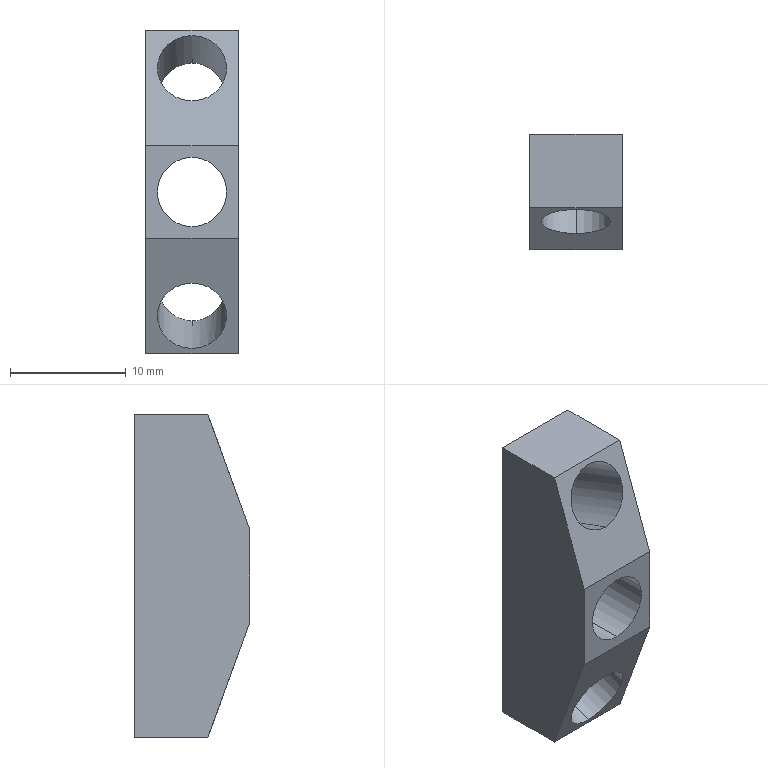Component | SolidWorks | ConnectingBlock-1 | 1 solid | 14 faces | box 8 x 10 x 28 mm | volume 1211 mm3 | plane 8 | cylinder 6 | commonest cylinder face diameters 6 x6
STEP:
#1=CARTESIAN_POINT('',(-5.544,0.8852,39.537));
#2=VERTEX_POINT('',#1);
#3=CARTESIAN_POINT('',(-5.544,0.8852,39.285));
#4=VERTEX_POINT('',#3);
#5=CARTESIAN_POINT('',(-5.544,0.8852,39.537));
#6=CARTESIAN_POINT('',(-5.308,0.8852,39.537));
#7=CARTESIAN_POINT('',(-5.308,0.8852,39.285));
#8=CARTESIAN_POINT('',(-5.544,0.8852,39.285));
#9=(BOUNDED_CURVE()B_SPLINE_CURVE(3,(#5,#6,#7,#8),.UNSPECIFIED.,.F.,.F.)B_SPLINE_CURVE_WITH_KNOTS((4,4),(3.142,6.283),.UNSPECIFIED.)CURVE()GEOMETRIC_REPRESENTATION_ITEM()RATIONAL_B_SPLINE_CURVE((1.,0.3333,0.3333,1.))REPRESENTATION_ITEM(''));
#10=EDGE_CURVE('',#2,#4,#9,.T.);
#11=ORIENTED_EDGE('',*,*,#10,.T.);
#12=CARTESIAN_POINT('',(-5.544,0.628,39.192));
#13=VERTEX_POINT('',#12);
#14=CARTESIAN_POINT('',(-5.544,1.109,39.367));
#15=DIRECTION('',(-0.,-0.9397,-0.342));
#16=VECTOR('',#15,39.37);
#17=LINE('',#14,#16);
#18=EDGE_CURVE('',#4,#13,#17,.T.);
#19=ORIENTED_EDGE('',*,*,#18,.T.);
#20=CARTESIAN_POINT('',(-5.544,0.5472,39.414));
#21=VERTEX_POINT('',#20);
#22=CARTESIAN_POINT('',(-5.544,0.5876,39.303));
#23=DIRECTION('',(0.,0.9397,0.342));
#24=DIRECTION('',(0.,0.342,-0.9397));
#25=AXIS2_PLACEMENT_3D('',#22,#23,#24);
#26=CIRCLE('',#25,0.1181);
#27=EDGE_CURVE('',#21,#13,#26,.T.);
#28=ORIENTED_EDGE('',*,*,#27,.F.);
#29=CARTESIAN_POINT('',(-5.544,1.028,39.589));
#30=DIRECTION('',(-0.,-0.9397,-0.342));
#31=VECTOR('',#30,39.37);
#32=LINE('',#29,#31);
#33=EDGE_CURVE('',#2,#21,#32,.T.);
#34=ORIENTED_EDGE('',*,*,#33,.F.);
#35=EDGE_LOOP('',(#11,#19,#28,#34));
#36=FACE_OUTER_BOUND('',#35,.T.);
#37=CARTESIAN_POINT('',(-5.544,1.069,39.478));
#38=DIRECTION('',(-0.,-0.9397,-0.342));
#39=DIRECTION('',(0.,-0.342,0.9397));
#40=AXIS2_PLACEMENT_3D('',#37,#38,#39);
#41=CYLINDRICAL_SURFACE('',#40,0.1181);
#42=ADVANCED_FACE('',(#36),#41,.F.);
#43=CARTESIAN_POINT('',(-5.544,0.8852,39.912));
#44=VERTEX_POINT('',#43);
#45=CARTESIAN_POINT('',(-5.544,0.8852,40.164));
#46=VERTEX_POINT('',#45);
#47=CARTESIAN_POINT('',(-5.544,0.8852,39.912));
#48=CARTESIAN_POINT('',(-5.308,0.8852,39.912));
#49=CARTESIAN_POINT('',(-5.308,0.8852,40.164));
#50=CARTESIAN_POINT('',(-5.544,0.8852,40.164));
#51=(BOUNDED_CURVE()B_SPLINE_CURVE(3,(#47,#48,#49,#50),.UNSPECIFIED.,.F.,.F.)B_SPLINE_CURVE_WITH_KNOTS((4,4),(3.142,6.283),.UNSPECIFIED.)CURVE()GEOMETRIC_REPRESENTATION_ITEM()RATIONAL_B_SPLINE_CURVE((1.,0.3333,0.3333,1.))REPRESENTATION_ITEM(''));
#52=EDGE_CURVE('',#44,#46,#51,.T.);
#53=ORIENTED_EDGE('',*,*,#52,.F.);
#54=CARTESIAN_POINT('',(-5.544,0.5472,40.035));
#55=VERTEX_POINT('',#54);
#56=CARTESIAN_POINT('',(-5.544,1.028,39.86));
#57=DIRECTION('',(-0.,-0.9397,0.342));
#58=VECTOR('',#57,39.37);
#59=LINE('',#56,#58);
#60=EDGE_CURVE('',#44,#55,#59,.T.);
#61=ORIENTED_EDGE('',*,*,#60,.T.);
#62=CARTESIAN_POINT('',(-5.544,0.628,40.257));
#63=VERTEX_POINT('',#62);
#64=CARTESIAN_POINT('',(-5.544,0.5876,40.146));
#65=DIRECTION('',(-0.,-0.9397,0.342));
#66=DIRECTION('',(0.,0.342,0.9397));
#67=AXIS2_PLACEMENT_3D('',#64,#65,#66);
#68=CIRCLE('',#67,0.1181);
#69=EDGE_CURVE('',#55,#63,#68,.T.);
#70=ORIENTED_EDGE('',*,*,#69,.T.);
#71=CARTESIAN_POINT('',(-5.544,1.109,40.082));
#72=DIRECTION('',(-0.,-0.9397,0.342));
#73=VECTOR('',#72,39.37);
#74=LINE('',#71,#73);
#75=EDGE_CURVE('',#46,#63,#74,.T.);
#76=ORIENTED_EDGE('',*,*,#75,.F.);
#77=EDGE_LOOP('',(#53,#61,#70,#76));
#78=FACE_OUTER_BOUND('',#77,.T.);
#79=CARTESIAN_POINT('',(-5.544,1.069,39.971));
#80=DIRECTION('',(-0.,-0.9397,0.342));
#81=DIRECTION('',(0.,0.342,0.9397));
#82=AXIS2_PLACEMENT_3D('',#79,#80,#81);
#83=CYLINDRICAL_SURFACE('',#82,0.1181);
#84=ADVANCED_FACE('',(#78),#83,.F.);
#85=CARTESIAN_POINT('',(-5.544,0.8852,39.606));
#86=VERTEX_POINT('',#85);
#87=CARTESIAN_POINT('',(-5.544,0.8852,39.843));
#88=VERTEX_POINT('',#87);
#89=CARTESIAN_POINT('',(-5.544,0.8852,39.724));
#90=DIRECTION('',(-0.,-1.,0.));
#91=DIRECTION('',(0.,0.,1.));
#92=AXIS2_PLACEMENT_3D('',#89,#90,#91);
#93=CIRCLE('',#92,0.1181);
#94=EDGE_CURVE('',#86,#88,#93,.T.);
#95=ORIENTED_EDGE('',*,*,#94,.F.);
#96=CARTESIAN_POINT('',(-5.544,0.4915,39.606));
#97=VERTEX_POINT('',#96);
#98=CARTESIAN_POINT('',(-5.544,1.003,39.606));
#99=DIRECTION('',(-0.,-1.,0.));
#100=VECTOR('',#99,39.37);
#101=LINE('',#98,#100);
#102=EDGE_CURVE('',#86,#97,#101,.T.);
#103=ORIENTED_EDGE('',*,*,#102,.T.);
#104=CARTESIAN_POINT('',(-5.544,0.4915,39.843));
#105=VERTEX_POINT('',#104);
#106=CARTESIAN_POINT('',(-5.544,0.4915,39.724));
#107=DIRECTION('',(-0.,-1.,0.));
#108=DIRECTION('',(0.,0.,1.));
#109=AXIS2_PLACEMENT_3D('',#106,#107,#108);
#110=CIRCLE('',#109,0.1181);
#111=EDGE_CURVE('',#97,#105,#110,.T.);
#112=ORIENTED_EDGE('',*,*,#111,.T.);
#113=CARTESIAN_POINT('',(-5.544,1.003,39.843));
#114=DIRECTION('',(-0.,-1.,0.));
#115=VECTOR('',#114,39.37);
#116=LINE('',#113,#115);
#117=EDGE_CURVE('',#88,#105,#116,.T.);
#118=ORIENTED_EDGE('',*,*,#117,.F.);
#119=EDGE_LOOP('',(#95,#103,#112,#118));
#120=FACE_OUTER_BOUND('',#119,.T.);
#121=CARTESIAN_POINT('',(-5.544,1.003,39.724));
#122=DIRECTION('',(-0.,-1.,0.));
#123=DIRECTION('',(0.,0.,1.));
#124=AXIS2_PLACEMENT_3D('',#121,#122,#123);
#125=CYLINDRICAL_SURFACE('',#124,0.1181);
#126=ADVANCED_FACE('',(#120),#125,.F.);
#127=CARTESIAN_POINT('',(-5.387,0.8852,39.173));
#128=VERTEX_POINT('',#127);
#129=CARTESIAN_POINT('',(-5.387,0.6348,39.173));
#130=VERTEX_POINT('',#129);
#131=CARTESIAN_POINT('',(-5.387,0.6348,39.173));
#132=DIRECTION('',(-0.,-1.,0.));
#133=VECTOR('',#132,39.37);
#134=LINE('',#131,#133);
#135=EDGE_CURVE('',#128,#130,#134,.T.);
#136=ORIENTED_EDGE('',*,*,#135,.T.);
#137=CARTESIAN_POINT('',(-5.701,0.6348,39.173));
#138=VERTEX_POINT('',#137);
#139=CARTESIAN_POINT('',(-5.701,0.6348,39.173));
#140=DIRECTION('',(1.,-0.,-0.));
#141=VECTOR('',#140,39.37);
#142=LINE('',#139,#141);
#143=EDGE_CURVE('',#138,#130,#142,.T.);
#144=ORIENTED_EDGE('',*,*,#143,.F.);
#145=CARTESIAN_POINT('',(-5.701,0.8852,39.173));
#146=VERTEX_POINT('',#145);
#147=CARTESIAN_POINT('',(-5.701,0.6348,39.173));
#148=DIRECTION('',(-0.,-1.,0.));
#149=VECTOR('',#148,39.37);
#150=LINE('',#147,#149);
#151=EDGE_CURVE('',#146,#138,#150,.T.);
#152=ORIENTED_EDGE('',*,*,#151,.F.);
#153=CARTESIAN_POINT('',(-5.701,0.8852,39.173));
#154=DIRECTION('',(1.,-0.,-0.));
#155=VECTOR('',#154,39.37);
#156=LINE('',#153,#155);
#157=EDGE_CURVE('',#146,#128,#156,.T.);
#158=ORIENTED_EDGE('',*,*,#157,.T.);
#159=EDGE_LOOP('',(#136,#144,#152,#158));
#160=FACE_OUTER_BOUND('',#159,.T.);
#161=CARTESIAN_POINT('',(-5.701,0.6348,39.173));
#162=DIRECTION('',(0.,0.,1.));
#163=DIRECTION('',(0.,1.,-0.));
#164=AXIS2_PLACEMENT_3D('',#161,#162,#163);
#165=PLANE('',#164);
#166=ADVANCED_FACE('',(#160),#165,.F.);
#167=ORIENTED_EDGE('',*,*,#27,.T.);
#168=CARTESIAN_POINT('',(-5.544,0.5876,39.303));
#169=DIRECTION('',(0.,0.9397,0.342));
#170=DIRECTION('',(0.,0.342,-0.9397));
#171=AXIS2_PLACEMENT_3D('',#168,#169,#170);
#172=CIRCLE('',#171,0.1181);
#173=EDGE_CURVE('',#13,#21,#172,.T.);
#174=ORIENTED_EDGE('',*,*,#173,.T.);
#175=EDGE_LOOP('',(#167,#174));
#176=FACE_BOUND('',#175,.T.);
#177=CARTESIAN_POINT('',(-5.387,0.4915,39.567));
#178=VERTEX_POINT('',#177);
#179=CARTESIAN_POINT('',(-5.387,0.4915,39.567));
#180=DIRECTION('',(0.,-0.342,0.9397));
#181=VECTOR('',#180,39.37);
#182=LINE('',#179,#181);
#183=EDGE_CURVE('',#130,#178,#182,.T.);
#184=ORIENTED_EDGE('',*,*,#183,.T.);
#185=CARTESIAN_POINT('',(-5.701,0.4915,39.567));
#186=VERTEX_POINT('',#185);
#187=CARTESIAN_POINT('',(-5.701,0.4915,39.567));
#188=DIRECTION('',(1.,-0.,-0.));
#189=VECTOR('',#188,39.37);
#190=LINE('',#187,#189);
#191=EDGE_CURVE('',#186,#178,#190,.T.);
#192=ORIENTED_EDGE('',*,*,#191,.F.);
#193=CARTESIAN_POINT('',(-5.701,0.4915,39.567));
#194=DIRECTION('',(0.,-0.342,0.9397));
#195=VECTOR('',#194,39.37);
#196=LINE('',#193,#195);
#197=EDGE_CURVE('',#138,#186,#196,.T.);
#198=ORIENTED_EDGE('',*,*,#197,.F.);
#199=ORIENTED_EDGE('',*,*,#143,.T.);
#200=EDGE_LOOP('',(#184,#192,#198,#199));
#201=FACE_OUTER_BOUND('',#200,.T.);
#202=CARTESIAN_POINT('',(-5.701,0.4915,39.567));
#203=DIRECTION('',(0.,0.9397,0.342));
#204=DIRECTION('',(-0.,0.342,-0.9397));
#205=AXIS2_PLACEMENT_3D('',#202,#203,#204);
#206=PLANE('',#205);
#207=ADVANCED_FACE('',(#176,#201),#206,.F.);
#208=CARTESIAN_POINT('',(-5.544,0.4915,39.724));
#209=DIRECTION('',(-0.,-1.,0.));
#210=DIRECTION('',(0.,0.,1.));
#211=AXIS2_PLACEMENT_3D('',#208,#209,#210);
#212=CIRCLE('',#211,0.1181);
#213=EDGE_CURVE('',#105,#97,#212,.T.);
#214=ORIENTED_EDGE('',*,*,#213,.F.);
#215=ORIENTED_EDGE('',*,*,#111,.F.);
#216=EDGE_LOOP('',(#214,#215));
#217=FACE_BOUND('',#216,.T.);
#218=CARTESIAN_POINT('',(-5.387,0.4915,39.882));
#219=VERTEX_POINT('',#218);
#220=CARTESIAN_POINT('',(-5.387,0.4915,39.882));
#221=DIRECTION('',(0.,0.,1.));
#222=VECTOR('',#221,39.37);
#223=LINE('',#220,#222);
#224=EDGE_CURVE('',#178,#219,#223,.T.);
#225=ORIENTED_EDGE('',*,*,#224,.T.);
#226=CARTESIAN_POINT('',(-5.701,0.4915,39.882));
#227=VERTEX_POINT('',#226);
#228=CARTESIAN_POINT('',(-5.701,0.4915,39.882));
#229=DIRECTION('',(1.,-0.,-0.));
#230=VECTOR('',#229,39.37);
#231=LINE('',#228,#230);
#232=EDGE_CURVE('',#227,#219,#231,.T.);
#233=ORIENTED_EDGE('',*,*,#232,.F.);
#234=CARTESIAN_POINT('',(-5.701,0.4915,39.882));
#235=DIRECTION('',(0.,0.,1.));
#236=VECTOR('',#235,39.37);
#237=LINE('',#234,#236);
#238=EDGE_CURVE('',#186,#227,#237,.T.);
#239=ORIENTED_EDGE('',*,*,#238,.F.);
#240=ORIENTED_EDGE('',*,*,#191,.T.);
#241=EDGE_LOOP('',(#225,#233,#239,#240));
#242=FACE_OUTER_BOUND('',#241,.T.);
#243=CARTESIAN_POINT('',(-5.701,0.4915,39.882));
#244=DIRECTION('',(0.,1.,-0.));
#245=DIRECTION('',(-0.,-0.,-1.));
#246=AXIS2_PLACEMENT_3D('',#243,#244,#245);
#247=PLANE('',#246);
#248=ADVANCED_FACE('',(#217,#242),#247,.F.);
#249=CARTESIAN_POINT('',(-5.544,0.5876,40.146));
#250=DIRECTION('',(-0.,-0.9397,0.342));
#251=DIRECTION('',(0.,0.342,0.9397));
#252=AXIS2_PLACEMENT_3D('',#249,#250,#251);
#253=CIRCLE('',#252,0.1181);
#254=EDGE_CURVE('',#63,#55,#253,.T.);
#255=ORIENTED_EDGE('',*,*,#254,.F.);
#256=ORIENTED_EDGE('',*,*,#69,.F.);
#257=EDGE_LOOP('',(#255,#256));
#258=FACE_BOUND('',#257,.T.);
#259=CARTESIAN_POINT('',(-5.387,0.6348,40.276));
#260=VERTEX_POINT('',#259);
#261=CARTESIAN_POINT('',(-5.387,0.6348,40.276));
#262=DIRECTION('',(0.,0.342,0.9397));
#263=VECTOR('',#262,39.37);
#264=LINE('',#261,#263);
#265=EDGE_CURVE('',#219,#260,#264,.T.);
#266=ORIENTED_EDGE('',*,*,#265,.T.);
#267=CARTESIAN_POINT('',(-5.701,0.6348,40.276));
#268=VERTEX_POINT('',#267);
#269=CARTESIAN_POINT('',(-5.701,0.6348,40.276));
#270=DIRECTION('',(1.,-0.,-0.));
#271=VECTOR('',#270,39.37);
#272=LINE('',#269,#271);
#273=EDGE_CURVE('',#268,#260,#272,.T.);
#274=ORIENTED_EDGE('',*,*,#273,.F.);
#275=CARTESIAN_POINT('',(-5.701,0.6348,40.276));
#276=DIRECTION('',(0.,0.342,0.9397));
#277=VECTOR('',#276,39.37);
#278=LINE('',#275,#277);
#279=EDGE_CURVE('',#227,#268,#278,.T.);
#280=ORIENTED_EDGE('',*,*,#279,.F.);
#281=ORIENTED_EDGE('',*,*,#232,.T.);
#282=EDGE_LOOP('',(#266,#274,#280,#281));
#283=FACE_OUTER_BOUND('',#282,.T.);
#284=CARTESIAN_POINT('',(-5.701,0.6348,40.276));
#285=DIRECTION('',(0.,0.9397,-0.342));
#286=DIRECTION('',(-0.,-0.342,-0.9397));
#287=AXIS2_PLACEMENT_3D('',#284,#285,#286);
#288=PLANE('',#287);
#289=ADVANCED_FACE('',(#258,#283),#288,.F.);
#290=CARTESIAN_POINT('',(-5.387,0.8852,40.276));
#291=VERTEX_POINT('',#290);
#292=CARTESIAN_POINT('',(-5.387,0.8852,40.276));
#293=DIRECTION('',(0.,1.,-0.));
#294=VECTOR('',#293,39.37);
#295=LINE('',#292,#294);
#296=EDGE_CURVE('',#260,#291,#295,.T.);
#297=ORIENTED_EDGE('',*,*,#296,.T.);
#298=CARTESIAN_POINT('',(-5.701,0.8852,40.276));
#299=VERTEX_POINT('',#298);
#300=CARTESIAN_POINT('',(-5.701,0.8852,40.276));
#301=DIRECTION('',(1.,-0.,-0.));
#302=VECTOR('',#301,39.37);
#303=LINE('',#300,#302);
#304=EDGE_CURVE('',#299,#291,#303,.T.);
#305=ORIENTED_EDGE('',*,*,#304,.F.);
#306=CARTESIAN_POINT('',(-5.701,0.8852,40.276));
#307=DIRECTION('',(0.,1.,-0.));
#308=VECTOR('',#307,39.37);
#309=LINE('',#306,#308);
#310=EDGE_CURVE('',#268,#299,#309,.T.);
#311=ORIENTED_EDGE('',*,*,#310,.F.);
#312=ORIENTED_EDGE('',*,*,#273,.T.);
#313=EDGE_LOOP('',(#297,#305,#311,#312));
#314=FACE_OUTER_BOUND('',#313,.T.);
#315=CARTESIAN_POINT('',(-5.701,0.8852,40.276));
#316=DIRECTION('',(-0.,-0.,-1.));
#317=DIRECTION('',(1.,-0.,-0.));
#318=AXIS2_PLACEMENT_3D('',#315,#316,#317);
#319=PLANE('',#318);
#320=ADVANCED_FACE('',(#314),#319,.F.);
#321=ORIENTED_EDGE('',*,*,#10,.F.);
#322=CARTESIAN_POINT('',(-5.544,0.8852,39.285));
#323=CARTESIAN_POINT('',(-5.78,0.8852,39.285));
#324=CARTESIAN_POINT('',(-5.78,0.8852,39.537));
#325=CARTESIAN_POINT('',(-5.544,0.8852,39.537));
#326=(BOUNDED_CURVE()B_SPLINE_CURVE(3,(#322,#323,#324,#325),.UNSPECIFIED.,.F.,.F.)B_SPLINE_CURVE_WITH_KNOTS((4,4),(0.,3.142),.UNSPECIFIED.)CURVE()GEOMETRIC_REPRESENTATION_ITEM()RATIONAL_B_SPLINE_CURVE((1.,0.3333,0.3333,1.))REPRESENTATION_ITEM(''));
#327=EDGE_CURVE('',#4,#2,#326,.T.);
#328=ORIENTED_EDGE('',*,*,#327,.F.);
#329=EDGE_LOOP('',(#321,#328));
#330=FACE_BOUND('',#329,.T.);
#331=CARTESIAN_POINT('',(-5.544,0.8852,40.164));
#332=CARTESIAN_POINT('',(-5.78,0.8852,40.164));
#333=CARTESIAN_POINT('',(-5.78,0.8852,39.912));
#334=CARTESIAN_POINT('',(-5.544,0.8852,39.912));
#335=(BOUNDED_CURVE()B_SPLINE_CURVE(3,(#331,#332,#333,#334),.UNSPECIFIED.,.F.,.F.)B_SPLINE_CURVE_WITH_KNOTS((4,4),(0.,3.142),.UNSPECIFIED.)CURVE()GEOMETRIC_REPRESENTATION_ITEM()RATIONAL_B_SPLINE_CURVE((1.,0.3333,0.3333,1.))REPRESENTATION_ITEM(''));
#336=EDGE_CURVE('',#46,#44,#335,.T.);
#337=ORIENTED_EDGE('',*,*,#336,.T.);
#338=ORIENTED_EDGE('',*,*,#52,.T.);
#339=EDGE_LOOP('',(#337,#338));
#340=FACE_BOUND('',#339,.T.);
#341=CARTESIAN_POINT('',(-5.544,0.8852,39.724));
#342=DIRECTION('',(-0.,-1.,0.));
#343=DIRECTION('',(0.,0.,1.));
#344=AXIS2_PLACEMENT_3D('',#341,#342,#343);
#345=CIRCLE('',#344,0.1181);
#346=EDGE_CURVE('',#88,#86,#345,.T.);
#347=ORIENTED_EDGE('',*,*,#346,.T.);
#348=ORIENTED_EDGE('',*,*,#94,.T.);
#349=EDGE_LOOP('',(#347,#348));
#350=FACE_BOUND('',#349,.T.);
#351=CARTESIAN_POINT('',(-5.387,0.8852,40.276));
#352=DIRECTION('',(-0.,-0.,-1.));
#353=VECTOR('',#352,39.37);
#354=LINE('',#351,#353);
#355=EDGE_CURVE('',#291,#128,#354,.T.);
#356=ORIENTED_EDGE('',*,*,#355,.T.);
#357=ORIENTED_EDGE('',*,*,#157,.F.);
#358=CARTESIAN_POINT('',(-5.701,0.8852,40.276));
#359=DIRECTION('',(-0.,-0.,-1.));
#360=VECTOR('',#359,39.37);
#361=LINE('',#358,#360);
#362=EDGE_CURVE('',#299,#146,#361,.T.);
#363=ORIENTED_EDGE('',*,*,#362,.F.);
#364=ORIENTED_EDGE('',*,*,#304,.T.);
#365=EDGE_LOOP('',(#356,#357,#363,#364));
#366=FACE_OUTER_BOUND('',#365,.T.);
#367=CARTESIAN_POINT('',(-5.701,0.8852,40.276));
#368=DIRECTION('',(-0.,-1.,0.));
#369=DIRECTION('',(0.,0.,1.));
#370=AXIS2_PLACEMENT_3D('',#367,#368,#369);
#371=PLANE('',#370);
#372=ADVANCED_FACE('',(#330,#340,#350,#366),#371,.F.);
#373=ORIENTED_EDGE('',*,*,#151,.T.);
#374=ORIENTED_EDGE('',*,*,#197,.T.);
#375=ORIENTED_EDGE('',*,*,#238,.T.);
#376=ORIENTED_EDGE('',*,*,#279,.T.);
#377=ORIENTED_EDGE('',*,*,#310,.T.);
#378=ORIENTED_EDGE('',*,*,#362,.T.);
#379=EDGE_LOOP('',(#373,#374,#375,#376,#377,#378));
#380=FACE_OUTER_BOUND('',#379,.T.);
#381=CARTESIAN_POINT('',(-5.701,0.6348,40.276));
#382=DIRECTION('',(-1.,0.,0.));
#383=DIRECTION('',(-0.,-0.,-1.));
#384=AXIS2_PLACEMENT_3D('',#381,#382,#383);
#385=PLANE('',#384);
#386=ADVANCED_FACE('',(#380),#385,.T.);
#387=ORIENTED_EDGE('',*,*,#135,.F.);
#388=ORIENTED_EDGE('',*,*,#355,.F.);
#389=ORIENTED_EDGE('',*,*,#296,.F.);
#390=ORIENTED_EDGE('',*,*,#265,.F.);
#391=ORIENTED_EDGE('',*,*,#224,.F.);
#392=ORIENTED_EDGE('',*,*,#183,.F.);
#393=EDGE_LOOP('',(#387,#388,#389,#390,#391,#392));
#394=FACE_OUTER_BOUND('',#393,.T.);
#395=CARTESIAN_POINT('',(-5.387,0.6348,40.276));
#396=DIRECTION('',(-1.,0.,0.));
#397=DIRECTION('',(-0.,-0.,-1.));
#398=AXIS2_PLACEMENT_3D('',#395,#396,#397);
#399=PLANE('',#398);
#400=ADVANCED_FACE('',(#394),#399,.F.);
#401=ORIENTED_EDGE('',*,*,#102,.F.);
#402=ORIENTED_EDGE('',*,*,#346,.F.);
#403=ORIENTED_EDGE('',*,*,#117,.T.);
#404=ORIENTED_EDGE('',*,*,#213,.T.);
#405=EDGE_LOOP('',(#401,#402,#403,#404));
#406=FACE_OUTER_BOUND('',#405,.T.);
#407=CARTESIAN_POINT('',(-5.544,1.003,39.724));
#408=DIRECTION('',(-0.,-1.,0.));
#409=DIRECTION('',(0.,0.,1.));
#410=AXIS2_PLACEMENT_3D('',#407,#408,#409);
#411=CYLINDRICAL_SURFACE('',#410,0.1181);
#412=ADVANCED_FACE('',(#406),#411,.F.);
#413=ORIENTED_EDGE('',*,*,#60,.F.);
#414=ORIENTED_EDGE('',*,*,#336,.F.);
#415=ORIENTED_EDGE('',*,*,#75,.T.);
#416=ORIENTED_EDGE('',*,*,#254,.T.);
#417=EDGE_LOOP('',(#413,#414,#415,#416));
#418=FACE_OUTER_BOUND('',#417,.T.);
#419=CARTESIAN_POINT('',(-5.544,1.069,39.971));
#420=DIRECTION('',(-0.,-0.9397,0.342));
#421=DIRECTION('',(0.,0.342,0.9397));
#422=AXIS2_PLACEMENT_3D('',#419,#420,#421);
#423=CYLINDRICAL_SURFACE('',#422,0.1181);
#424=ADVANCED_FACE('',(#418),#423,.F.);
#425=ORIENTED_EDGE('',*,*,#18,.F.);
#426=ORIENTED_EDGE('',*,*,#327,.T.);
#427=ORIENTED_EDGE('',*,*,#33,.T.);
#428=ORIENTED_EDGE('',*,*,#173,.F.);
#429=EDGE_LOOP('',(#425,#426,#427,#428));
#430=FACE_OUTER_BOUND('',#429,.T.);
#431=CARTESIAN_POINT('',(-5.544,1.069,39.478));
#432=DIRECTION('',(-0.,-0.9397,-0.342));
#433=DIRECTION('',(0.,-0.342,0.9397));
#434=AXIS2_PLACEMENT_3D('',#431,#432,#433);
#435=CYLINDRICAL_SURFACE('',#434,0.1181);
#436=ADVANCED_FACE('',(#430),#435,.F.);
#437=CLOSED_SHELL('',(#42,#84,#126,#166,#207,#248,#289,#320,#372,#386,#400,#412,#424,#436));
#438=MANIFOLD_SOLID_BREP('',#437);
#439=CARTESIAN_POINT('',(0.,0.,0.));
#440=DIRECTION('',(0.,0.,1.));
#441=DIRECTION('',(1.,0.,0.));
#442=AXIS2_PLACEMENT_3D('',#439,#440,#441);
#443=(LENGTH_UNIT()NAMED_UNIT(*)SI_UNIT($,.METRE.));
#444=LENGTH_MEASURE_WITH_UNIT(LENGTH_MEASURE(0.0254),#443);
#445=DIMENSIONAL_EXPONENTS(1.,0.,0.,0.,0.,0.,0.);
#446=(CONVERSION_BASED_UNIT('',#444)LENGTH_UNIT()NAMED_UNIT(#445));
#447=UNCERTAINTY_MEASURE_WITH_UNIT(LENGTH_MEASURE(0.00001),#446,'','');
#448=(NAMED_UNIT(*)PLANE_ANGLE_UNIT()SI_UNIT($,.RADIAN.));
#449=(NAMED_UNIT(*)SI_UNIT($,.STERADIAN.)SOLID_ANGLE_UNIT());
#450=(GEOMETRIC_REPRESENTATION_CONTEXT(3)GLOBAL_UNCERTAINTY_ASSIGNED_CONTEXT((#447))GLOBAL_UNIT_ASSIGNED_CONTEXT((#446,#448,#449))REPRESENTATION_CONTEXT('',''));
#451=ADVANCED_BREP_SHAPE_REPRESENTATION('',(#438,#442),#450);
#452=COLOUR_RGB('',0.7922,0.8196,0.9333);
#453=FILL_AREA_STYLE_COLOUR('',#452);
#454=FILL_AREA_STYLE('',(#453));
#455=SURFACE_STYLE_FILL_AREA(#454);
#456=SURFACE_SIDE_STYLE('',(#455));
#457=SURFACE_STYLE_USAGE(.BOTH.,#456);
#458=PRESENTATION_STYLE_ASSIGNMENT((#457));
#459=STYLED_ITEM('',(#458),#438);
#460=(LENGTH_UNIT()NAMED_UNIT(*)SI_UNIT($,.METRE.));
#461=LENGTH_MEASURE_WITH_UNIT(LENGTH_MEASURE(0.0254),#460);
#462=DIMENSIONAL_EXPONENTS(1.,0.,0.,0.,0.,0.,0.);
#463=(CONVERSION_BASED_UNIT('',#461)LENGTH_UNIT()NAMED_UNIT(#462));
#464=UNCERTAINTY_MEASURE_WITH_UNIT(LENGTH_MEASURE(0.00001),#463,'','');
#465=(NAMED_UNIT(*)PLANE_ANGLE_UNIT()SI_UNIT($,.RADIAN.));
#466=(NAMED_UNIT(*)SI_UNIT($,.STERADIAN.)SOLID_ANGLE_UNIT());
#467=(GEOMETRIC_REPRESENTATION_CONTEXT(3)GLOBAL_UNCERTAINTY_ASSIGNED_CONTEXT((#464))GLOBAL_UNIT_ASSIGNED_CONTEXT((#463,#465,#466))REPRESENTATION_CONTEXT('',''));
#468=MECHANICAL_DESIGN_GEOMETRIC_PRESENTATION_REPRESENTATION('',(#459),#467);
#469=PRESENTATION_LAYER_ASSIGNMENT('','',(#459));